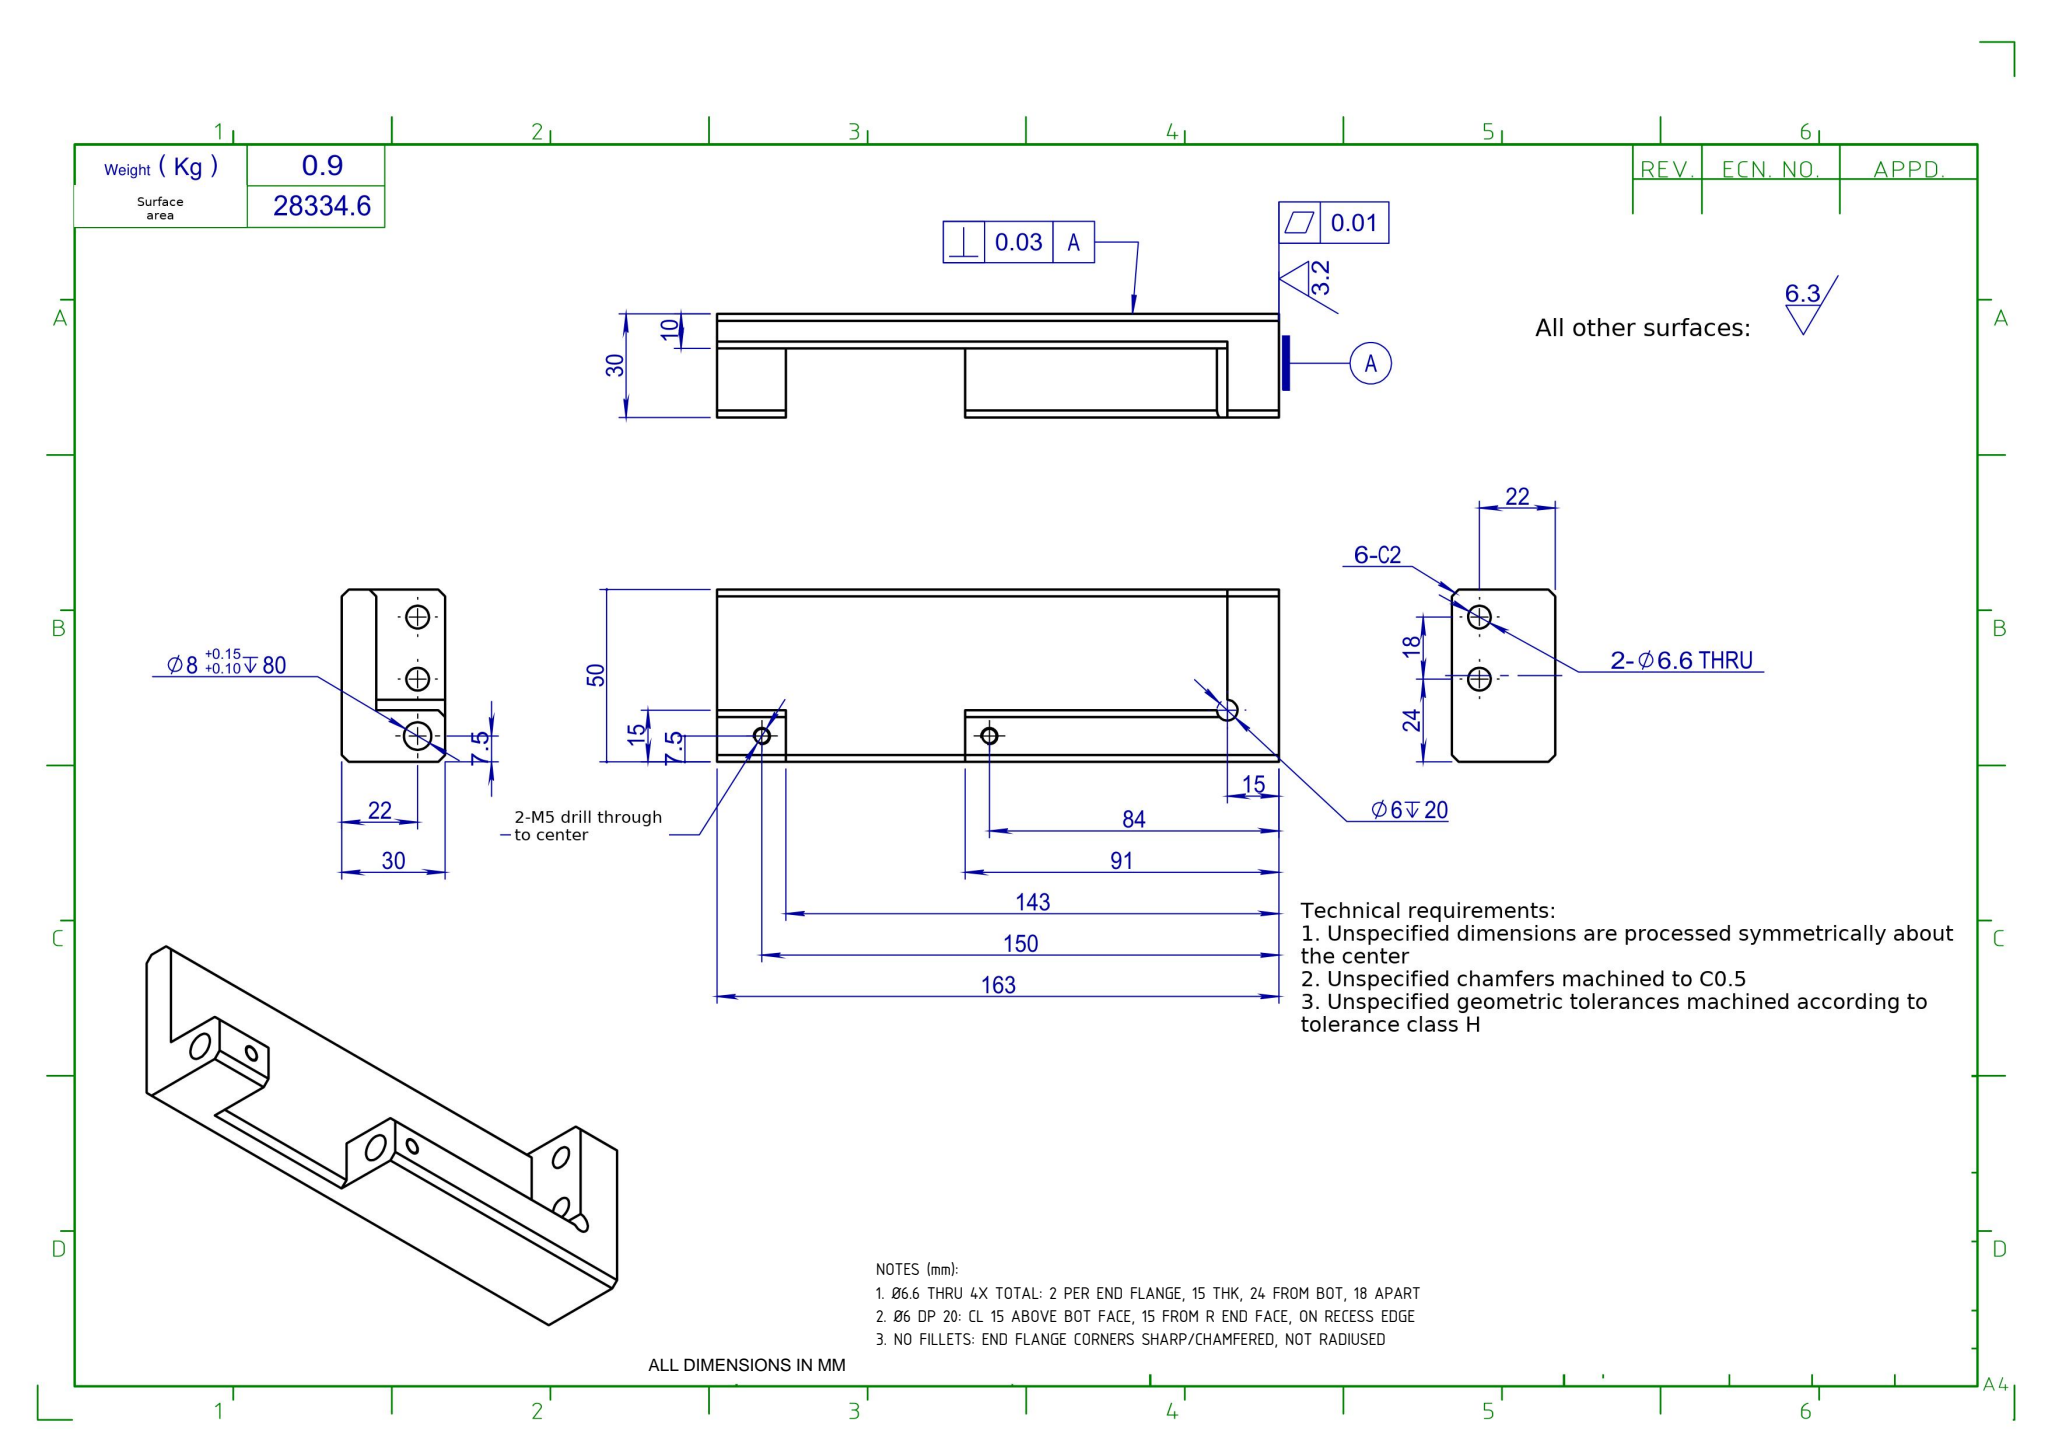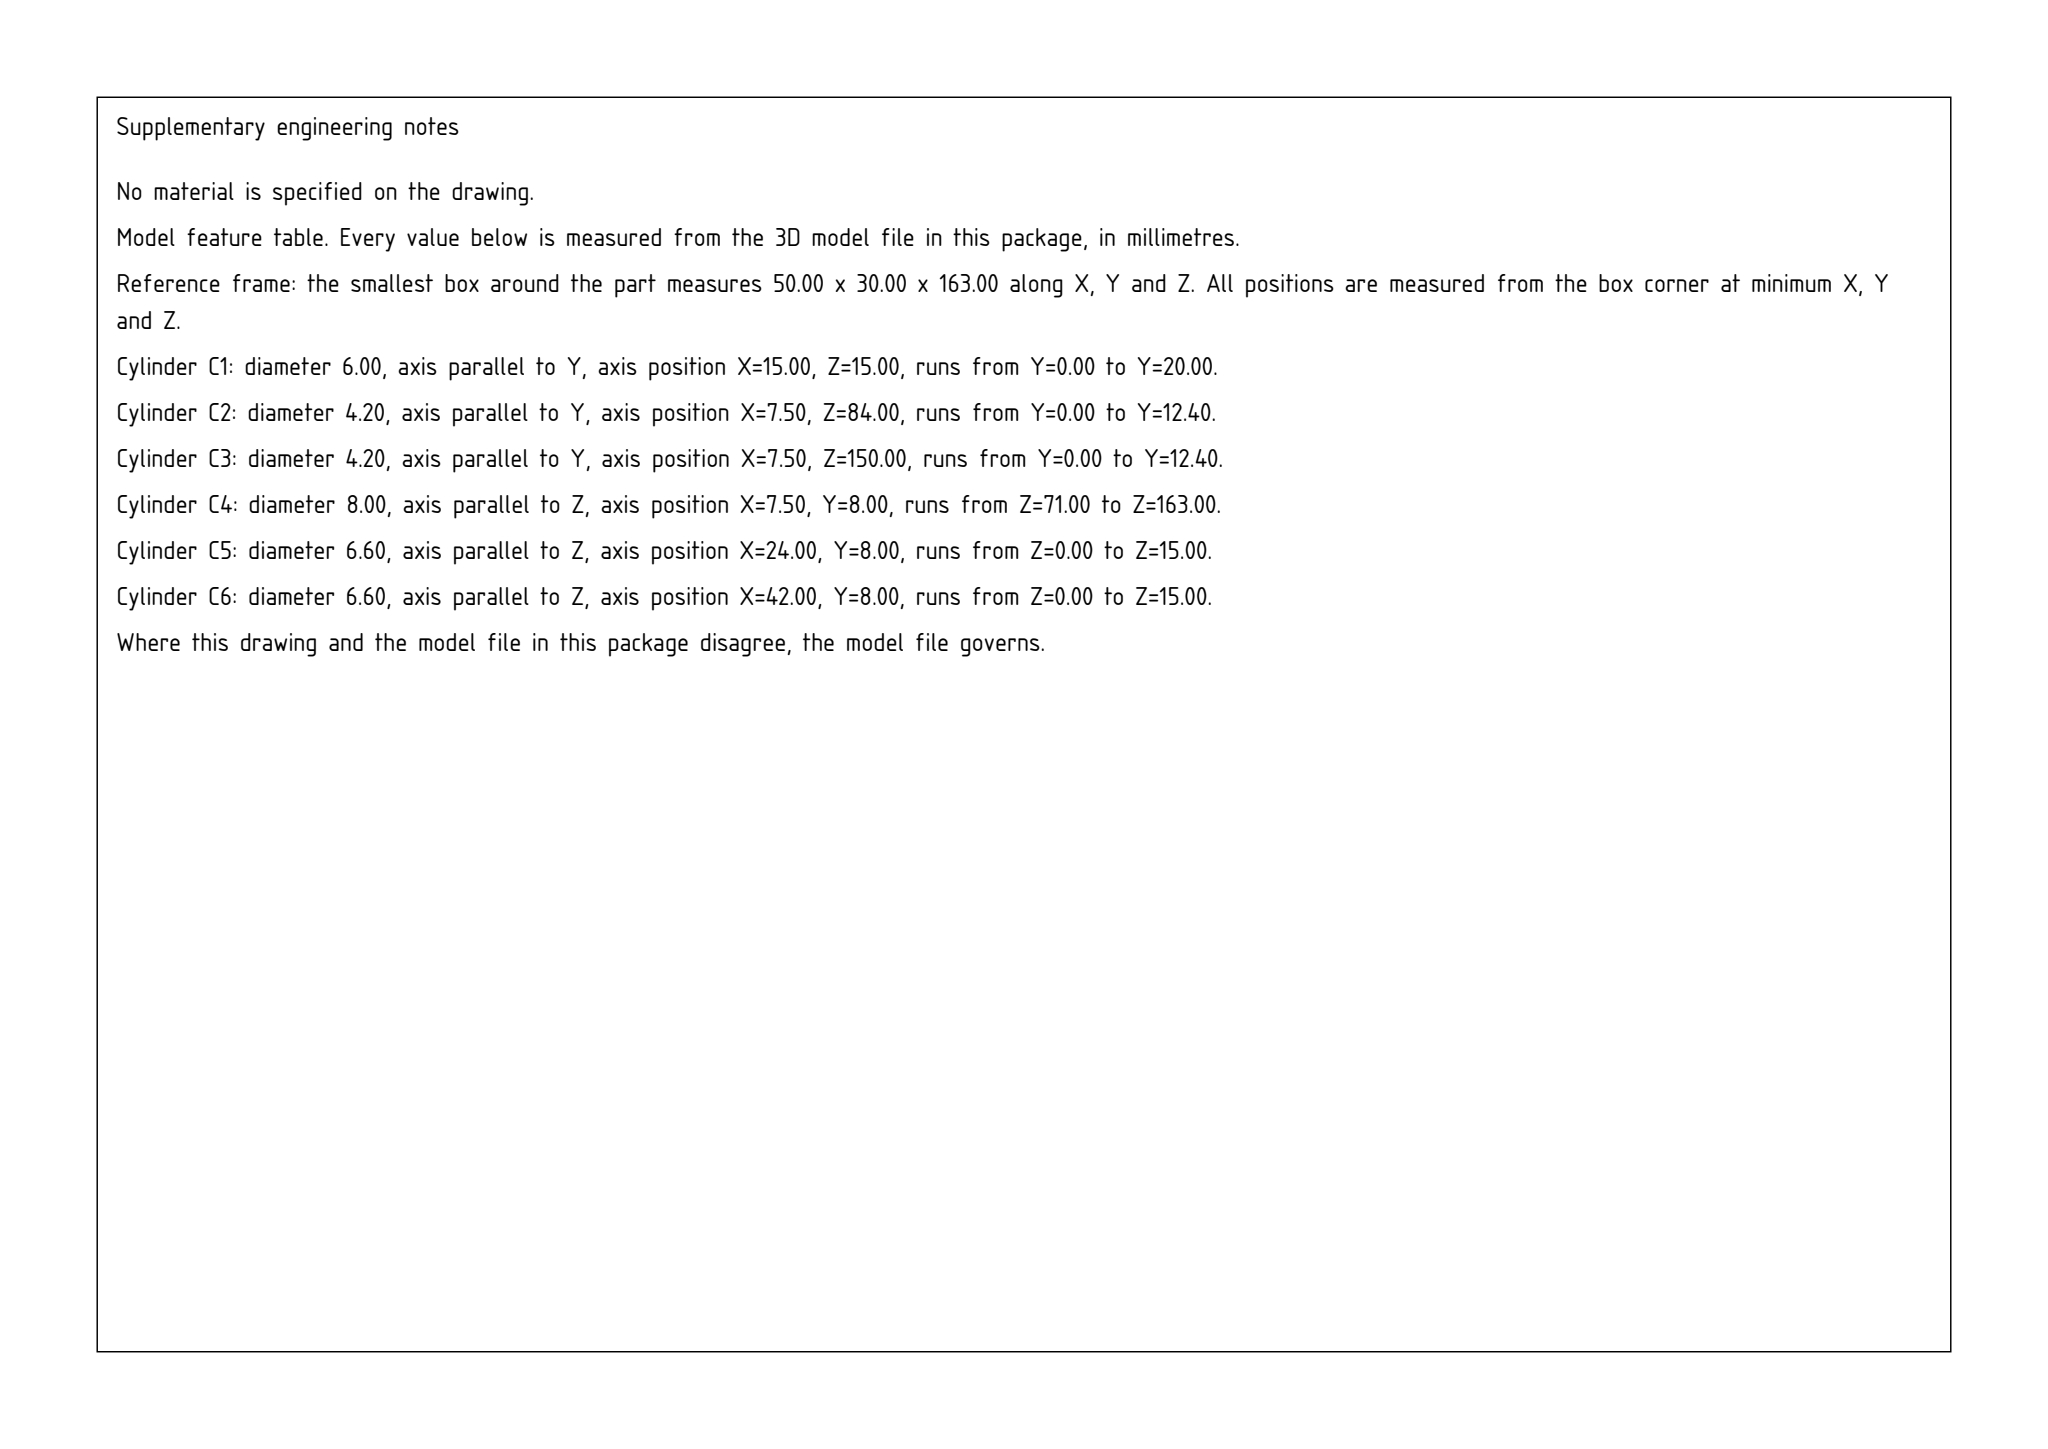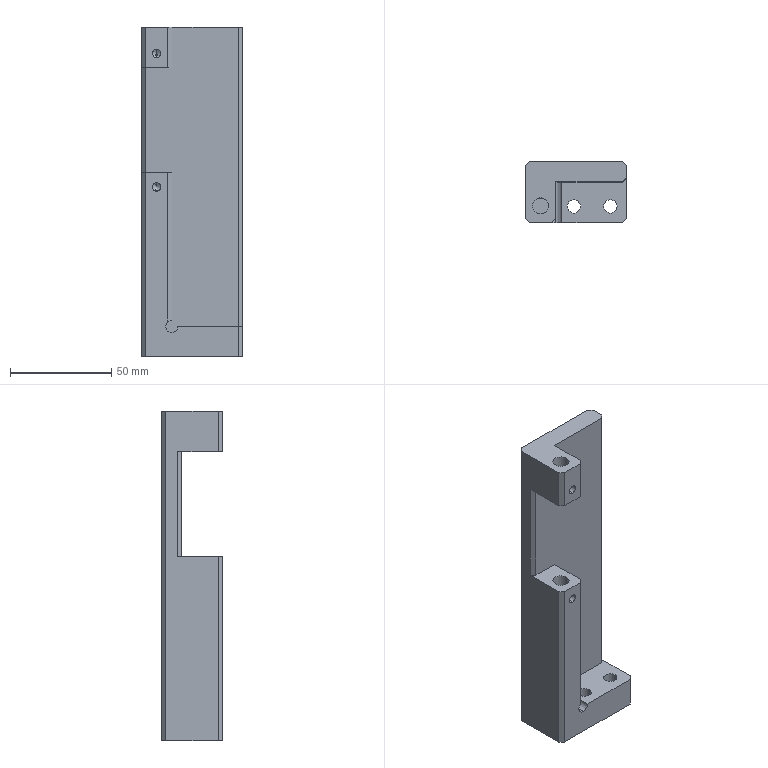Part | SolidWorks | mm | 1 solid | 45 faces | box 50 x 30 x 163 mm | volume 120207 mm3 | plane 23 | cylinder 18 | cone 4 | commonest cylinder face diameters 4.2 x8 8 x4 6.6 x4 6 x2
Drawing notes:
Ø6.6 THRU 4X TOTAL: 2 PER END FLANGE, 15 THK, 24 FROM BOT, 18 APART | from the solid: 6.6 dia z-axis cyls at x=24 and x=42, y=8, len 15, count 2 each (both end flanges)
Ø6 DP 20: CL 15 ABOVE BOT FACE, 15 FROM R END FACE, ON RECESS EDGE | from the solid: cylinder dia 6.0, axis y, pos [x=15.0, z=15.0], depth 20; z-normal plane at offset 15.0
NO FILLETS: END FLANGE CORNERS SHARP/CHAMFERED, NOT RADIUSED | from the solid: fillet_radii: [] - model contains no fillet surfaces
build123d program:
from build123d import *

# Parameters (mm, degrees)
SKETCH1_W             = 50
SKETCH1_H             = 30
EXTRUDE1_DEPTH        = 7.5
SKETCH2_W             = 50
SKETCH2_H             = 10
EXTRUDE2_DEPTH        = 148
SKETCH3_W             = 148
SKETCH3_H             = 30
EXTRUDE3_DEPTH        = 15
SKETCH4_R             = 3.3
CUT_EXTRUDE1_DEPTH    = 151.844
SKETCH5_W             = 15
SKETCH5_H             = 52
CUT_EXTRUDE2_DEPTH    = 20
SKETCH6_R             = 4
CUT_EXTRUDE3_DEPTH    = 92
SKETCH15_R            = 3
CUT_EXTRUDE5_DEPTH    = 20
CHAMFER1_SIZE         = 2
M5_TAPPED_HOLE1_D     = 4.2
M5_TAPPED_HOLE1_DEPTH = 12.4
M5_TAPPED_HOLE1_TIP   = 1.262


with BuildPart() as part:
    # Sketch1 → Extrude1 (new, symmetric)
    with BuildSketch(Plane.XY):
        Rectangle(SKETCH1_W, SKETCH1_H)
    extrude(amount=EXTRUDE1_DEPTH, both=True)

    # Sketch2 → Extrude2 (add)
    with BuildSketch(Plane.XY.offset(7.5)):
        with Locations((0, 10)):
            Rectangle(SKETCH2_W, SKETCH2_H)
    extrude(amount=EXTRUDE2_DEPTH)

    # Sketch3 → Extrude3 (add)
    with BuildSketch(Plane(origin=(-25, 0, 0), x_dir=(0, 0, -1), z_dir=(1, 0, 0))):
        with Locations((-81.5, 0)):
            Rectangle(SKETCH3_W, SKETCH3_H)
    extrude(amount=EXTRUDE3_DEPTH)

    # Sketch4 → Cut-Extrude1 (cut, through all)
    with BuildSketch(Plane.XY.offset(7.5)):
        with Locations((17, -7)):
            Circle(SKETCH4_R)
        with Locations(Location((-1, -7, 0), (0, 0, 180))):
            Circle(SKETCH4_R)
    extrude(amount=-CUT_EXTRUDE1_DEPTH, mode=Mode.SUBTRACT)

    # Sketch5 → Cut-Extrude2 (cut)
    with BuildSketch(Plane(origin=(0, -15, 0), x_dir=(1, 0, 0), z_dir=(0, 1, 0))):
        with Locations((-17.5, -109.5)):
            Rectangle(SKETCH5_W, SKETCH5_H)
    extrude(amount=CUT_EXTRUDE2_DEPTH, mode=Mode.SUBTRACT)

    # Sketch6 → Cut-Extrude3 (cut)
    with BuildSketch(Plane.XY.offset(155.5)):
        with Locations((-17.5, -7)):
            Circle(SKETCH6_R)
    extrude(amount=-CUT_EXTRUDE3_DEPTH, mode=Mode.SUBTRACT)

    # Sketch15 → Cut-Extrude5 (cut)
    with BuildSketch(Plane.XZ.offset(15)):
        with Locations((-10, 7.5)):
            Circle(SKETCH15_R)
    extrude(amount=-CUT_EXTRUDE5_DEPTH, mode=Mode.SUBTRACT)

    # Chamfer1
    chamfer1_edges = [part.edges().sort_by_distance(p)[0] for p in [
        (-25, -15, 145.5),
        (-25, -15, 38),
        (-25, 15, 74),
        (25, -15, 0),
        (-25, 5, 109.5),
        (25, 15, 74),
        (25, 5, 81.5),
        (-10, -15, 47),
        (-10, -15, 145.5),
    ]]
    chamfer(chamfer1_edges, length=CHAMFER1_SIZE)

    # M5 Tapped Hole1
    with Locations(Plane.XZ.offset(15)):
        with Locations((-17.5, 76.5), (-17.5, 142.5)):
            Hole(M5_TAPPED_HOLE1_D / 2, depth=M5_TAPPED_HOLE1_DEPTH)
            with Locations((0, 0, -(M5_TAPPED_HOLE1_DEPTH + M5_TAPPED_HOLE1_TIP / 2))):  # 118° drill point
                Cone(0, M5_TAPPED_HOLE1_D / 2, M5_TAPPED_HOLE1_TIP, mode=Mode.SUBTRACT)


solid = part.part